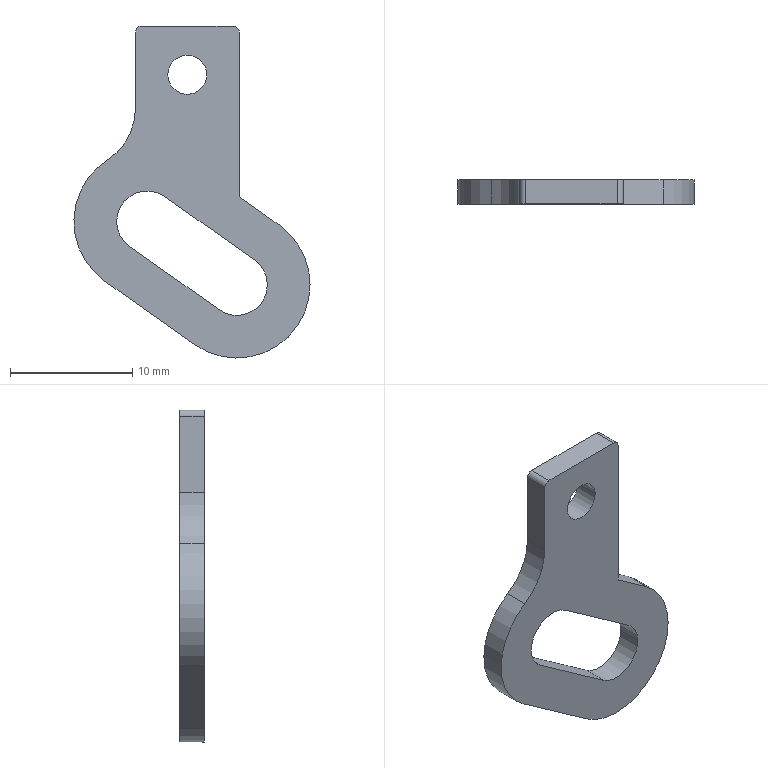Component | SolidWorks | CLS-MechanismOperatingAxisBracketAssembly.SLDPRT-1_CLS-MechanismPositioningSlide-1 | 1 solid | 20 faces | box 19.35 x 2 x 27.21 mm | volume 493 mm3 | cylinder 11 | plane 9 | commonest cylinder face diameters 5 x3 12 x3 3.2 x2 1 x2 10 x1
STEP:
#1=COLOUR_RGB('',0.7922,0.8196,0.9333);
#2=FILL_AREA_STYLE_COLOUR('',#1);
#3=FILL_AREA_STYLE('',(#2));
#4=SURFACE_STYLE_FILL_AREA(#3);
#5=SURFACE_SIDE_STYLE('',(#4));
#6=SURFACE_STYLE_USAGE(.BOTH.,#5);
#7=PRESENTATION_STYLE_ASSIGNMENT((#6));
#8=CARTESIAN_POINT('',(-2.391,-0.8783,-2.185));
#9=VERTEX_POINT('',#8);
#10=CARTESIAN_POINT('',(-2.265,-0.8783,-2.185));
#11=VERTEX_POINT('',#10);
#12=CARTESIAN_POINT('',(-2.328,-0.8783,-2.185));
#13=DIRECTION('',(0.,1.,-0.));
#14=DIRECTION('',(1.,0.,0.));
#15=AXIS2_PLACEMENT_3D('',#12,#13,#14);
#16=CIRCLE('',#15,0.06299);
#17=EDGE_CURVE('',#9,#11,#16,.T.);
#18=ORIENTED_EDGE('',*,*,#17,.F.);
#19=CARTESIAN_POINT('',(-2.391,-0.7995,-2.185));
#20=VERTEX_POINT('',#19);
#21=CARTESIAN_POINT('',(-2.391,-0.8783,-2.185));
#22=DIRECTION('',(0.,1.,-0.));
#23=VECTOR('',#22,39.37);
#24=LINE('',#21,#23);
#25=EDGE_CURVE('',#9,#20,#24,.T.);
#26=ORIENTED_EDGE('',*,*,#25,.T.);
#27=CARTESIAN_POINT('',(-2.265,-0.7995,-2.185));
#28=VERTEX_POINT('',#27);
#29=CARTESIAN_POINT('',(-2.328,-0.7995,-2.185));
#30=DIRECTION('',(0.,1.,-0.));
#31=DIRECTION('',(1.,0.,0.));
#32=AXIS2_PLACEMENT_3D('',#29,#30,#31);
#33=CIRCLE('',#32,0.06299);
#34=EDGE_CURVE('',#20,#28,#33,.T.);
#35=ORIENTED_EDGE('',*,*,#34,.T.);
#36=CARTESIAN_POINT('',(-2.265,-0.8783,-2.185));
#37=DIRECTION('',(0.,1.,-0.));
#38=VECTOR('',#37,39.37);
#39=LINE('',#36,#38);
#40=EDGE_CURVE('',#11,#28,#39,.T.);
#41=ORIENTED_EDGE('',*,*,#40,.F.);
#42=EDGE_LOOP('',(#18,#26,#35,#41));
#43=FACE_OUTER_BOUND('',#42,.T.);
#44=CARTESIAN_POINT('',(-2.328,-0.8783,-2.185));
#45=DIRECTION('',(0.,1.,-0.));
#46=DIRECTION('',(1.,0.,0.));
#47=AXIS2_PLACEMENT_3D('',#44,#45,#46);
#48=CYLINDRICAL_SURFACE('',#47,0.06299);
#49=ADVANCED_FACE('',(#43),#48,.F.);
#50=CARTESIAN_POINT('',(-2.07,-0.8783,-2.862));
#51=VERTEX_POINT('',#50);
#52=CARTESIAN_POINT('',(-2.225,-0.8783,-2.943));
#53=VERTEX_POINT('',#52);
#54=CARTESIAN_POINT('',(-2.168,-0.8783,-2.862));
#55=DIRECTION('',(0.,1.,-0.));
#56=DIRECTION('',(1.,0.,0.));
#57=AXIS2_PLACEMENT_3D('',#54,#55,#56);
#58=CIRCLE('',#57,0.09843);
#59=EDGE_CURVE('',#51,#53,#58,.T.);
#60=ORIENTED_EDGE('',*,*,#59,.F.);
#61=CARTESIAN_POINT('',(-2.07,-0.7995,-2.862));
#62=VERTEX_POINT('',#61);
#63=CARTESIAN_POINT('',(-2.07,-0.8783,-2.862));
#64=DIRECTION('',(0.,1.,-0.));
#65=VECTOR('',#64,39.37);
#66=LINE('',#63,#65);
#67=EDGE_CURVE('',#51,#62,#66,.T.);
#68=ORIENTED_EDGE('',*,*,#67,.T.);
#69=CARTESIAN_POINT('',(-2.225,-0.7995,-2.943));
#70=VERTEX_POINT('',#69);
#71=CARTESIAN_POINT('',(-2.168,-0.7995,-2.862));
#72=DIRECTION('',(0.,1.,-0.));
#73=DIRECTION('',(1.,0.,0.));
#74=AXIS2_PLACEMENT_3D('',#71,#72,#73);
#75=CIRCLE('',#74,0.09843);
#76=EDGE_CURVE('',#62,#70,#75,.T.);
#77=ORIENTED_EDGE('',*,*,#76,.T.);
#78=CARTESIAN_POINT('',(-2.225,-0.8783,-2.943));
#79=DIRECTION('',(0.,1.,-0.));
#80=VECTOR('',#79,39.37);
#81=LINE('',#78,#80);
#82=EDGE_CURVE('',#53,#70,#81,.T.);
#83=ORIENTED_EDGE('',*,*,#82,.F.);
#84=EDGE_LOOP('',(#60,#68,#77,#83));
#85=FACE_OUTER_BOUND('',#84,.T.);
#86=CARTESIAN_POINT('',(-2.168,-0.8783,-2.862));
#87=DIRECTION('',(0.,1.,-0.));
#88=DIRECTION('',(1.,0.,0.));
#89=AXIS2_PLACEMENT_3D('',#86,#87,#88);
#90=CYLINDRICAL_SURFACE('',#89,0.09843);
#91=ADVANCED_FACE('',(#85),#90,.F.);
#92=CARTESIAN_POINT('',(-2.032,-0.8783,-2.669));
#93=VERTEX_POINT('',#92);
#94=CARTESIAN_POINT('',(-1.932,-0.8783,-2.862));
#95=VERTEX_POINT('',#94);
#96=CARTESIAN_POINT('',(-2.168,-0.8783,-2.862));
#97=DIRECTION('',(0.,1.,-0.));
#98=DIRECTION('',(1.,0.,0.));
#99=AXIS2_PLACEMENT_3D('',#96,#97,#98);
#100=CIRCLE('',#99,0.2362);
#101=EDGE_CURVE('',#93,#95,#100,.T.);
#102=ORIENTED_EDGE('',*,*,#101,.T.);
#103=CARTESIAN_POINT('',(-1.932,-0.7995,-2.862));
#104=VERTEX_POINT('',#103);
#105=CARTESIAN_POINT('',(-1.932,-0.8783,-2.862));
#106=DIRECTION('',(0.,1.,-0.));
#107=VECTOR('',#106,39.37);
#108=LINE('',#105,#107);
#109=EDGE_CURVE('',#95,#104,#108,.T.);
#110=ORIENTED_EDGE('',*,*,#109,.T.);
#111=CARTESIAN_POINT('',(-2.032,-0.7995,-2.669));
#112=VERTEX_POINT('',#111);
#113=CARTESIAN_POINT('',(-2.168,-0.7995,-2.862));
#114=DIRECTION('',(0.,1.,-0.));
#115=DIRECTION('',(1.,0.,0.));
#116=AXIS2_PLACEMENT_3D('',#113,#114,#115);
#117=CIRCLE('',#116,0.2362);
#118=EDGE_CURVE('',#112,#104,#117,.T.);
#119=ORIENTED_EDGE('',*,*,#118,.F.);
#120=CARTESIAN_POINT('',(-2.032,-0.8783,-2.669));
#121=DIRECTION('',(0.,1.,-0.));
#122=VECTOR('',#121,39.37);
#123=LINE('',#120,#122);
#124=EDGE_CURVE('',#93,#112,#123,.T.);
#125=ORIENTED_EDGE('',*,*,#124,.F.);
#126=EDGE_LOOP('',(#102,#110,#119,#125));
#127=FACE_OUTER_BOUND('',#126,.T.);
#128=CARTESIAN_POINT('',(-2.168,-0.8783,-2.862));
#129=DIRECTION('',(0.,1.,-0.));
#130=DIRECTION('',(1.,0.,0.));
#131=AXIS2_PLACEMENT_3D('',#128,#129,#130);
#132=CYLINDRICAL_SURFACE('',#131,0.2362);
#133=ADVANCED_FACE('',(#127),#132,.T.);
#134=CARTESIAN_POINT('',(-2.495,-0.8783,-2.294));
#135=VERTEX_POINT('',#134);
#136=CARTESIAN_POINT('',(-2.495,-0.8783,-2.047));
#137=VERTEX_POINT('',#136);
#138=CARTESIAN_POINT('',(-2.495,-0.8783,-2.425));
#139=DIRECTION('',(0.,0.,1.));
#140=VECTOR('',#139,39.37);
#141=LINE('',#138,#140);
#142=EDGE_CURVE('',#135,#137,#141,.T.);
#143=ORIENTED_EDGE('',*,*,#142,.T.);
#144=CARTESIAN_POINT('',(-2.495,-0.7995,-2.047));
#145=VERTEX_POINT('',#144);
#146=CARTESIAN_POINT('',(-2.495,-0.8783,-2.047));
#147=DIRECTION('',(0.,1.,-0.));
#148=VECTOR('',#147,39.37);
#149=LINE('',#146,#148);
#150=EDGE_CURVE('',#137,#145,#149,.T.);
#151=ORIENTED_EDGE('',*,*,#150,.T.);
#152=CARTESIAN_POINT('',(-2.495,-0.7995,-2.294));
#153=VERTEX_POINT('',#152);
#154=CARTESIAN_POINT('',(-2.495,-0.7995,-2.425));
#155=DIRECTION('',(0.,0.,1.));
#156=VECTOR('',#155,39.37);
#157=LINE('',#154,#156);
#158=EDGE_CURVE('',#153,#145,#157,.T.);
#159=ORIENTED_EDGE('',*,*,#158,.F.);
#160=CARTESIAN_POINT('',(-2.495,-0.8783,-2.294));
#161=DIRECTION('',(-0.,-1.,0.));
#162=VECTOR('',#161,39.37);
#163=LINE('',#160,#162);
#164=EDGE_CURVE('',#153,#135,#163,.T.);
#165=ORIENTED_EDGE('',*,*,#164,.T.);
#166=EDGE_LOOP('',(#143,#151,#159,#165));
#167=FACE_OUTER_BOUND('',#166,.T.);
#168=CARTESIAN_POINT('',(-2.495,-0.8783,-2.425));
#169=DIRECTION('',(-1.,0.,0.));
#170=DIRECTION('',(0.,1.,-0.));
#171=AXIS2_PLACEMENT_3D('',#168,#169,#170);
#172=PLANE('',#171);
#173=ADVANCED_FACE('',(#167),#172,.T.);
#174=CARTESIAN_POINT('',(-2.594,-0.8783,-2.851));
#175=VERTEX_POINT('',#174);
#176=CARTESIAN_POINT('',(-2.585,-0.8783,-2.459));
#177=VERTEX_POINT('',#176);
#178=CARTESIAN_POINT('',(-2.458,-0.8783,-2.658));
#179=DIRECTION('',(0.,1.,-0.));
#180=DIRECTION('',(1.,0.,0.));
#181=AXIS2_PLACEMENT_3D('',#178,#179,#180);
#182=CIRCLE('',#181,0.2362);
#183=EDGE_CURVE('',#175,#177,#182,.T.);
#184=ORIENTED_EDGE('',*,*,#183,.T.);
#185=CARTESIAN_POINT('',(-2.585,-0.7995,-2.459));
#186=VERTEX_POINT('',#185);
#187=CARTESIAN_POINT('',(-2.585,-0.8783,-2.459));
#188=DIRECTION('',(0.,1.,-0.));
#189=VECTOR('',#188,39.37);
#190=LINE('',#187,#189);
#191=EDGE_CURVE('',#177,#186,#190,.T.);
#192=ORIENTED_EDGE('',*,*,#191,.T.);
#193=CARTESIAN_POINT('',(-2.594,-0.7995,-2.851));
#194=VERTEX_POINT('',#193);
#195=CARTESIAN_POINT('',(-2.458,-0.7995,-2.658));
#196=DIRECTION('',(0.,1.,-0.));
#197=DIRECTION('',(1.,0.,0.));
#198=AXIS2_PLACEMENT_3D('',#195,#196,#197);
#199=CIRCLE('',#198,0.2362);
#200=EDGE_CURVE('',#194,#186,#199,.T.);
#201=ORIENTED_EDGE('',*,*,#200,.F.);
#202=CARTESIAN_POINT('',(-2.594,-0.8783,-2.851));
#203=DIRECTION('',(0.,1.,-0.));
#204=VECTOR('',#203,39.37);
#205=LINE('',#202,#204);
#206=EDGE_CURVE('',#175,#194,#205,.T.);
#207=ORIENTED_EDGE('',*,*,#206,.F.);
#208=EDGE_LOOP('',(#184,#192,#201,#207));
#209=FACE_OUTER_BOUND('',#208,.T.);
#210=CARTESIAN_POINT('',(-2.458,-0.8783,-2.658));
#211=DIRECTION('',(0.,1.,-0.));
#212=DIRECTION('',(1.,0.,0.));
#213=AXIS2_PLACEMENT_3D('',#210,#211,#212);
#214=CYLINDRICAL_SURFACE('',#213,0.2362);
#215=ADVANCED_FACE('',(#209),#214,.T.);
#216=CARTESIAN_POINT('',(-2.304,-0.7995,-3.055));
#217=VERTEX_POINT('',#216);
#218=CARTESIAN_POINT('',(-2.594,-0.7995,-2.851));
#219=DIRECTION('',(-0.817,0.,0.5767));
#220=VECTOR('',#219,39.37);
#221=LINE('',#218,#220);
#222=EDGE_CURVE('',#217,#194,#221,.T.);
#223=ORIENTED_EDGE('',*,*,#222,.F.);
#224=CARTESIAN_POINT('',(-2.304,-0.8783,-3.055));
#225=VERTEX_POINT('',#224);
#226=CARTESIAN_POINT('',(-2.304,-0.8783,-3.055));
#227=DIRECTION('',(0.,1.,-0.));
#228=VECTOR('',#227,39.37);
#229=LINE('',#226,#228);
#230=EDGE_CURVE('',#225,#217,#229,.T.);
#231=ORIENTED_EDGE('',*,*,#230,.F.);
#232=CARTESIAN_POINT('',(-2.594,-0.8783,-2.851));
#233=DIRECTION('',(-0.817,0.,0.5767));
#234=VECTOR('',#233,39.37);
#235=LINE('',#232,#234);
#236=EDGE_CURVE('',#225,#175,#235,.T.);
#237=ORIENTED_EDGE('',*,*,#236,.T.);
#238=ORIENTED_EDGE('',*,*,#206,.T.);
#239=EDGE_LOOP('',(#223,#231,#237,#238));
#240=FACE_OUTER_BOUND('',#239,.T.);
#241=CARTESIAN_POINT('',(-2.594,-0.8783,-2.851));
#242=DIRECTION('',(-0.5767,-0.,-0.817));
#243=DIRECTION('',(-0.817,0.,0.5767));
#244=AXIS2_PLACEMENT_3D('',#241,#242,#243);
#245=PLANE('',#244);
#246=ADVANCED_FACE('',(#240),#245,.T.);
#247=ORIENTED_EDGE('',*,*,#109,.F.);
#248=CARTESIAN_POINT('',(-2.168,-0.8783,-2.862));
#249=DIRECTION('',(0.,1.,-0.));
#250=DIRECTION('',(1.,0.,0.));
#251=AXIS2_PLACEMENT_3D('',#248,#249,#250);
#252=CIRCLE('',#251,0.2362);
#253=EDGE_CURVE('',#95,#225,#252,.T.);
#254=ORIENTED_EDGE('',*,*,#253,.T.);
#255=ORIENTED_EDGE('',*,*,#230,.T.);
#256=CARTESIAN_POINT('',(-2.168,-0.7995,-2.862));
#257=DIRECTION('',(0.,1.,-0.));
#258=DIRECTION('',(1.,0.,0.));
#259=AXIS2_PLACEMENT_3D('',#256,#257,#258);
#260=CIRCLE('',#259,0.2362);
#261=EDGE_CURVE('',#104,#217,#260,.T.);
#262=ORIENTED_EDGE('',*,*,#261,.F.);
#263=EDGE_LOOP('',(#247,#254,#255,#262));
#264=FACE_OUTER_BOUND('',#263,.T.);
#265=CARTESIAN_POINT('',(-2.168,-0.8783,-2.862));
#266=DIRECTION('',(0.,1.,-0.));
#267=DIRECTION('',(1.,0.,0.));
#268=AXIS2_PLACEMENT_3D('',#265,#266,#267);
#269=CYLINDRICAL_SURFACE('',#268,0.2362);
#270=ADVANCED_FACE('',(#264),#269,.T.);
#271=CARTESIAN_POINT('',(-2.161,-0.7995,-2.578));
#272=VERTEX_POINT('',#271);
#273=CARTESIAN_POINT('',(-2.161,-0.7995,-2.578));
#274=DIRECTION('',(0.817,-0.,-0.5767));
#275=VECTOR('',#274,39.37);
#276=LINE('',#273,#275);
#277=EDGE_CURVE('',#272,#112,#276,.T.);
#278=ORIENTED_EDGE('',*,*,#277,.F.);
#279=CARTESIAN_POINT('',(-2.161,-0.8783,-2.578));
#280=VERTEX_POINT('',#279);
#281=CARTESIAN_POINT('',(-2.161,-0.8783,-2.578));
#282=DIRECTION('',(0.,1.,-0.));
#283=VECTOR('',#282,39.37);
#284=LINE('',#281,#283);
#285=EDGE_CURVE('',#280,#272,#284,.T.);
#286=ORIENTED_EDGE('',*,*,#285,.F.);
#287=CARTESIAN_POINT('',(-2.161,-0.8783,-2.578));
#288=DIRECTION('',(0.817,-0.,-0.5767));
#289=VECTOR('',#288,39.37);
#290=LINE('',#287,#289);
#291=EDGE_CURVE('',#280,#93,#290,.T.);
#292=ORIENTED_EDGE('',*,*,#291,.T.);
#293=ORIENTED_EDGE('',*,*,#124,.T.);
#294=EDGE_LOOP('',(#278,#286,#292,#293));
#295=FACE_OUTER_BOUND('',#294,.T.);
#296=CARTESIAN_POINT('',(-2.161,-0.8783,-2.578));
#297=DIRECTION('',(0.5767,0.,0.817));
#298=DIRECTION('',(0.817,-0.,-0.5767));
#299=AXIS2_PLACEMENT_3D('',#296,#297,#298);
#300=PLANE('',#299);
#301=ADVANCED_FACE('',(#295),#300,.T.);
#302=CARTESIAN_POINT('',(-2.161,-0.7995,-2.047));
#303=VERTEX_POINT('',#302);
#304=CARTESIAN_POINT('',(-2.161,-0.7995,-2.027));
#305=DIRECTION('',(-0.,-0.,-1.));
#306=VECTOR('',#305,39.37);
#307=LINE('',#304,#306);
#308=EDGE_CURVE('',#303,#272,#307,.T.);
#309=ORIENTED_EDGE('',*,*,#308,.F.);
#310=CARTESIAN_POINT('',(-2.161,-0.8783,-2.047));
#311=VERTEX_POINT('',#310);
#312=CARTESIAN_POINT('',(-2.161,-0.8783,-2.047));
#313=DIRECTION('',(-0.,-1.,0.));
#314=VECTOR('',#313,39.37);
#315=LINE('',#312,#314);
#316=EDGE_CURVE('',#303,#311,#315,.T.);
#317=ORIENTED_EDGE('',*,*,#316,.T.);
#318=CARTESIAN_POINT('',(-2.161,-0.8783,-2.027));
#319=DIRECTION('',(-0.,-0.,-1.));
#320=VECTOR('',#319,39.37);
#321=LINE('',#318,#320);
#322=EDGE_CURVE('',#311,#280,#321,.T.);
#323=ORIENTED_EDGE('',*,*,#322,.T.);
#324=ORIENTED_EDGE('',*,*,#285,.T.);
#325=EDGE_LOOP('',(#309,#317,#323,#324));
#326=FACE_OUTER_BOUND('',#325,.T.);
#327=CARTESIAN_POINT('',(-2.161,-0.8783,-2.027));
#328=DIRECTION('',(1.,-0.,-0.));
#329=DIRECTION('',(-0.,-1.,0.));
#330=AXIS2_PLACEMENT_3D('',#327,#328,#329);
#331=PLANE('',#330);
#332=ADVANCED_FACE('',(#326),#331,.T.);
#333=CARTESIAN_POINT('',(-2.475,-0.7995,-2.027));
#334=VERTEX_POINT('',#333);
#335=CARTESIAN_POINT('',(-2.18,-0.7995,-2.027));
#336=VERTEX_POINT('',#335);
#337=CARTESIAN_POINT('',(-2.495,-0.7995,-2.027));
#338=DIRECTION('',(1.,-0.,-0.));
#339=VECTOR('',#338,39.37);
#340=LINE('',#337,#339);
#341=EDGE_CURVE('',#334,#336,#340,.T.);
#342=ORIENTED_EDGE('',*,*,#341,.F.);
#343=CARTESIAN_POINT('',(-2.475,-0.8783,-2.027));
#344=VERTEX_POINT('',#343);
#345=CARTESIAN_POINT('',(-2.475,-0.8783,-2.027));
#346=DIRECTION('',(-0.,-1.,0.));
#347=VECTOR('',#346,39.37);
#348=LINE('',#345,#347);
#349=EDGE_CURVE('',#334,#344,#348,.T.);
#350=ORIENTED_EDGE('',*,*,#349,.T.);
#351=CARTESIAN_POINT('',(-2.18,-0.8783,-2.027));
#352=VERTEX_POINT('',#351);
#353=CARTESIAN_POINT('',(-2.495,-0.8783,-2.027));
#354=DIRECTION('',(1.,-0.,-0.));
#355=VECTOR('',#354,39.37);
#356=LINE('',#353,#355);
#357=EDGE_CURVE('',#344,#352,#356,.T.);
#358=ORIENTED_EDGE('',*,*,#357,.T.);
#359=CARTESIAN_POINT('',(-2.18,-0.8783,-2.027));
#360=DIRECTION('',(0.,1.,-0.));
#361=VECTOR('',#360,39.37);
#362=LINE('',#359,#361);
#363=EDGE_CURVE('',#352,#336,#362,.T.);
#364=ORIENTED_EDGE('',*,*,#363,.T.);
#365=EDGE_LOOP('',(#342,#350,#358,#364));
#366=FACE_OUTER_BOUND('',#365,.T.);
#367=CARTESIAN_POINT('',(-2.495,-0.8783,-2.027));
#368=DIRECTION('',(0.,0.,1.));
#369=DIRECTION('',(-0.,-1.,0.));
#370=AXIS2_PLACEMENT_3D('',#367,#368,#369);
#371=PLANE('',#370);
#372=ADVANCED_FACE('',(#366),#371,.T.);
#373=CARTESIAN_POINT('',(-2.328,-0.8783,-2.185));
#374=DIRECTION('',(0.,1.,-0.));
#375=DIRECTION('',(1.,0.,0.));
#376=AXIS2_PLACEMENT_3D('',#373,#374,#375);
#377=CIRCLE('',#376,0.06299);
#378=EDGE_CURVE('',#11,#9,#377,.T.);
#379=ORIENTED_EDGE('',*,*,#378,.T.);
#380=ORIENTED_EDGE('',*,*,#17,.T.);
#381=EDGE_LOOP('',(#379,#380));
#382=FACE_BOUND('',#381,.T.);
#383=CARTESIAN_POINT('',(-2.514,-0.8783,-2.738));
#384=VERTEX_POINT('',#383);
#385=CARTESIAN_POINT('',(-2.401,-0.8783,-2.577));
#386=VERTEX_POINT('',#385);
#387=CARTESIAN_POINT('',(-2.458,-0.8783,-2.658));
#388=DIRECTION('',(0.,1.,-0.));
#389=DIRECTION('',(1.,0.,0.));
#390=AXIS2_PLACEMENT_3D('',#387,#388,#389);
#391=CIRCLE('',#390,0.09843);
#392=EDGE_CURVE('',#384,#386,#391,.T.);
#393=ORIENTED_EDGE('',*,*,#392,.T.);
#394=CARTESIAN_POINT('',(-2.111,-0.8783,-2.782));
#395=VERTEX_POINT('',#394);
#396=CARTESIAN_POINT('',(-2.111,-0.8783,-2.782));
#397=DIRECTION('',(0.817,-0.,-0.5767));
#398=VECTOR('',#397,39.37);
#399=LINE('',#396,#398);
#400=EDGE_CURVE('',#386,#395,#399,.T.);
#401=ORIENTED_EDGE('',*,*,#400,.T.);
#402=CARTESIAN_POINT('',(-2.168,-0.8783,-2.862));
#403=DIRECTION('',(0.,1.,-0.));
#404=DIRECTION('',(1.,0.,0.));
#405=AXIS2_PLACEMENT_3D('',#402,#403,#404);
#406=CIRCLE('',#405,0.09843);
#407=EDGE_CURVE('',#395,#51,#406,.T.);
#408=ORIENTED_EDGE('',*,*,#407,.T.);
#409=ORIENTED_EDGE('',*,*,#59,.T.);
#410=CARTESIAN_POINT('',(-2.225,-0.8783,-2.943));
#411=DIRECTION('',(-0.817,0.,0.5767));
#412=VECTOR('',#411,39.37);
#413=LINE('',#410,#412);
#414=EDGE_CURVE('',#53,#384,#413,.T.);
#415=ORIENTED_EDGE('',*,*,#414,.T.);
#416=EDGE_LOOP('',(#393,#401,#408,#409,#415));
#417=FACE_BOUND('',#416,.T.);
#418=ORIENTED_EDGE('',*,*,#357,.F.);
#419=CARTESIAN_POINT('',(-2.475,-0.8783,-2.047));
#420=DIRECTION('',(-0.,-1.,0.));
#421=DIRECTION('',(1.,0.,0.));
#422=AXIS2_PLACEMENT_3D('',#419,#420,#421);
#423=CIRCLE('',#422,0.01969);
#424=EDGE_CURVE('',#344,#137,#423,.T.);
#425=ORIENTED_EDGE('',*,*,#424,.T.);
#426=ORIENTED_EDGE('',*,*,#142,.F.);
#427=CARTESIAN_POINT('',(-2.692,-0.8783,-2.294));
#428=DIRECTION('',(0.,1.,-0.));
#429=DIRECTION('',(1.,0.,0.));
#430=AXIS2_PLACEMENT_3D('',#427,#428,#429);
#431=CIRCLE('',#430,0.1969);
#432=EDGE_CURVE('',#135,#177,#431,.T.);
#433=ORIENTED_EDGE('',*,*,#432,.T.);
#434=ORIENTED_EDGE('',*,*,#183,.F.);
#435=ORIENTED_EDGE('',*,*,#236,.F.);
#436=ORIENTED_EDGE('',*,*,#253,.F.);
#437=ORIENTED_EDGE('',*,*,#101,.F.);
#438=ORIENTED_EDGE('',*,*,#291,.F.);
#439=ORIENTED_EDGE('',*,*,#322,.F.);
#440=CARTESIAN_POINT('',(-2.18,-0.8783,-2.047));
#441=DIRECTION('',(-0.,-1.,0.));
#442=DIRECTION('',(1.,0.,0.));
#443=AXIS2_PLACEMENT_3D('',#440,#441,#442);
#444=CIRCLE('',#443,0.01969);
#445=EDGE_CURVE('',#311,#352,#444,.T.);
#446=ORIENTED_EDGE('',*,*,#445,.T.);
#447=EDGE_LOOP('',(#418,#425,#426,#433,#434,#435,#436,#437,#438,#439,#446));
#448=FACE_OUTER_BOUND('',#447,.T.);
#449=CARTESIAN_POINT('',(-2.168,-0.8783,-2.862));
#450=DIRECTION('',(0.,1.,-0.));
#451=DIRECTION('',(1.,-0.,-0.));
#452=AXIS2_PLACEMENT_3D('',#449,#450,#451);
#453=PLANE('',#452);
#454=ADVANCED_FACE('',(#382,#417,#448),#453,.F.);
#455=CARTESIAN_POINT('',(-2.328,-0.7995,-2.185));
#456=DIRECTION('',(0.,1.,-0.));
#457=DIRECTION('',(1.,0.,0.));
#458=AXIS2_PLACEMENT_3D('',#455,#456,#457);
#459=CIRCLE('',#458,0.06299);
#460=EDGE_CURVE('',#28,#20,#459,.T.);
#461=ORIENTED_EDGE('',*,*,#460,.F.);
#462=ORIENTED_EDGE('',*,*,#34,.F.);
#463=EDGE_LOOP('',(#461,#462));
#464=FACE_BOUND('',#463,.T.);
#465=CARTESIAN_POINT('',(-2.401,-0.7995,-2.577));
#466=VERTEX_POINT('',#465);
#467=CARTESIAN_POINT('',(-2.111,-0.7995,-2.782));
#468=VERTEX_POINT('',#467);
#469=CARTESIAN_POINT('',(-2.111,-0.7995,-2.782));
#470=DIRECTION('',(0.817,-0.,-0.5767));
#471=VECTOR('',#470,39.37);
#472=LINE('',#469,#471);
#473=EDGE_CURVE('',#466,#468,#472,.T.);
#474=ORIENTED_EDGE('',*,*,#473,.F.);
#475=CARTESIAN_POINT('',(-2.514,-0.7995,-2.738));
#476=VERTEX_POINT('',#475);
#477=CARTESIAN_POINT('',(-2.458,-0.7995,-2.658));
#478=DIRECTION('',(0.,1.,-0.));
#479=DIRECTION('',(1.,0.,0.));
#480=AXIS2_PLACEMENT_3D('',#477,#478,#479);
#481=CIRCLE('',#480,0.09843);
#482=EDGE_CURVE('',#476,#466,#481,.T.);
#483=ORIENTED_EDGE('',*,*,#482,.F.);
#484=CARTESIAN_POINT('',(-2.225,-0.7995,-2.943));
#485=DIRECTION('',(-0.817,0.,0.5767));
#486=VECTOR('',#485,39.37);
#487=LINE('',#484,#486);
#488=EDGE_CURVE('',#70,#476,#487,.T.);
#489=ORIENTED_EDGE('',*,*,#488,.F.);
#490=ORIENTED_EDGE('',*,*,#76,.F.);
#491=CARTESIAN_POINT('',(-2.168,-0.7995,-2.862));
#492=DIRECTION('',(0.,1.,-0.));
#493=DIRECTION('',(1.,0.,0.));
#494=AXIS2_PLACEMENT_3D('',#491,#492,#493);
#495=CIRCLE('',#494,0.09843);
#496=EDGE_CURVE('',#468,#62,#495,.T.);
#497=ORIENTED_EDGE('',*,*,#496,.F.);
#498=EDGE_LOOP('',(#474,#483,#489,#490,#497));
#499=FACE_BOUND('',#498,.T.);
#500=ORIENTED_EDGE('',*,*,#158,.T.);
#501=CARTESIAN_POINT('',(-2.475,-0.7995,-2.047));
#502=DIRECTION('',(0.,1.,-0.));
#503=DIRECTION('',(1.,0.,0.));
#504=AXIS2_PLACEMENT_3D('',#501,#502,#503);
#505=CIRCLE('',#504,0.01969);
#506=EDGE_CURVE('',#145,#334,#505,.T.);
#507=ORIENTED_EDGE('',*,*,#506,.T.);
#508=ORIENTED_EDGE('',*,*,#341,.T.);
#509=CARTESIAN_POINT('',(-2.18,-0.7995,-2.047));
#510=DIRECTION('',(0.,1.,-0.));
#511=DIRECTION('',(1.,0.,0.));
#512=AXIS2_PLACEMENT_3D('',#509,#510,#511);
#513=CIRCLE('',#512,0.01969);
#514=EDGE_CURVE('',#336,#303,#513,.T.);
#515=ORIENTED_EDGE('',*,*,#514,.T.);
#516=ORIENTED_EDGE('',*,*,#308,.T.);
#517=ORIENTED_EDGE('',*,*,#277,.T.);
#518=ORIENTED_EDGE('',*,*,#118,.T.);
#519=ORIENTED_EDGE('',*,*,#261,.T.);
#520=ORIENTED_EDGE('',*,*,#222,.T.);
#521=ORIENTED_EDGE('',*,*,#200,.T.);
#522=CARTESIAN_POINT('',(-2.692,-0.7995,-2.294));
#523=DIRECTION('',(-0.,-1.,0.));
#524=DIRECTION('',(1.,0.,0.));
#525=AXIS2_PLACEMENT_3D('',#522,#523,#524);
#526=CIRCLE('',#525,0.1969);
#527=EDGE_CURVE('',#186,#153,#526,.T.);
#528=ORIENTED_EDGE('',*,*,#527,.T.);
#529=EDGE_LOOP('',(#500,#507,#508,#515,#516,#517,#518,#519,#520,#521,#528));
#530=FACE_OUTER_BOUND('',#529,.T.);
#531=CARTESIAN_POINT('',(-2.168,-0.7995,-2.862));
#532=DIRECTION('',(0.,1.,-0.));
#533=DIRECTION('',(1.,-0.,-0.));
#534=AXIS2_PLACEMENT_3D('',#531,#532,#533);
#535=PLANE('',#534);
#536=ADVANCED_FACE('',(#464,#499,#530),#535,.T.);
#537=ORIENTED_EDGE('',*,*,#473,.T.);
#538=CARTESIAN_POINT('',(-2.111,-0.8783,-2.782));
#539=DIRECTION('',(0.,1.,-0.));
#540=VECTOR('',#539,39.37);
#541=LINE('',#538,#540);
#542=EDGE_CURVE('',#395,#468,#541,.T.);
#543=ORIENTED_EDGE('',*,*,#542,.F.);
#544=ORIENTED_EDGE('',*,*,#400,.F.);
#545=CARTESIAN_POINT('',(-2.401,-0.8783,-2.577));
#546=DIRECTION('',(0.,1.,-0.));
#547=VECTOR('',#546,39.37);
#548=LINE('',#545,#547);
#549=EDGE_CURVE('',#386,#466,#548,.T.);
#550=ORIENTED_EDGE('',*,*,#549,.T.);
#551=EDGE_LOOP('',(#537,#543,#544,#550));
#552=FACE_OUTER_BOUND('',#551,.T.);
#553=CARTESIAN_POINT('',(-2.111,-0.8783,-2.782));
#554=DIRECTION('',(0.5767,0.,0.817));
#555=DIRECTION('',(0.817,-0.,-0.5767));
#556=AXIS2_PLACEMENT_3D('',#553,#554,#555);
#557=PLANE('',#556);
#558=ADVANCED_FACE('',(#552),#557,.F.);
#559=ORIENTED_EDGE('',*,*,#482,.T.);
#560=ORIENTED_EDGE('',*,*,#549,.F.);
#561=ORIENTED_EDGE('',*,*,#392,.F.);
#562=CARTESIAN_POINT('',(-2.514,-0.8783,-2.738));
#563=DIRECTION('',(0.,1.,-0.));
#564=VECTOR('',#563,39.37);
#565=LINE('',#562,#564);
#566=EDGE_CURVE('',#384,#476,#565,.T.);
#567=ORIENTED_EDGE('',*,*,#566,.T.);
#568=EDGE_LOOP('',(#559,#560,#561,#567));
#569=FACE_OUTER_BOUND('',#568,.T.);
#570=CARTESIAN_POINT('',(-2.458,-0.8783,-2.658));
#571=DIRECTION('',(0.,1.,-0.));
#572=DIRECTION('',(1.,0.,0.));
#573=AXIS2_PLACEMENT_3D('',#570,#571,#572);
#574=CYLINDRICAL_SURFACE('',#573,0.09843);
#575=ADVANCED_FACE('',(#569),#574,.F.);
#576=ORIENTED_EDGE('',*,*,#488,.T.);
#577=ORIENTED_EDGE('',*,*,#566,.F.);
#578=ORIENTED_EDGE('',*,*,#414,.F.);
#579=ORIENTED_EDGE('',*,*,#82,.T.);
#580=EDGE_LOOP('',(#576,#577,#578,#579));
#581=FACE_OUTER_BOUND('',#580,.T.);
#582=CARTESIAN_POINT('',(-2.225,-0.8783,-2.943));
#583=DIRECTION('',(-0.5767,-0.,-0.817));
#584=DIRECTION('',(-0.817,0.,0.5767));
#585=AXIS2_PLACEMENT_3D('',#582,#583,#584);
#586=PLANE('',#585);
#587=ADVANCED_FACE('',(#581),#586,.F.);
#588=ORIENTED_EDGE('',*,*,#67,.F.);
#589=ORIENTED_EDGE('',*,*,#407,.F.);
#590=ORIENTED_EDGE('',*,*,#542,.T.);
#591=ORIENTED_EDGE('',*,*,#496,.T.);
#592=EDGE_LOOP('',(#588,#589,#590,#591));
#593=FACE_OUTER_BOUND('',#592,.T.);
#594=CARTESIAN_POINT('',(-2.168,-0.8783,-2.862));
#595=DIRECTION('',(0.,1.,-0.));
#596=DIRECTION('',(1.,0.,0.));
#597=AXIS2_PLACEMENT_3D('',#594,#595,#596);
#598=CYLINDRICAL_SURFACE('',#597,0.09843);
#599=ADVANCED_FACE('',(#593),#598,.F.);
#600=ORIENTED_EDGE('',*,*,#432,.F.);
#601=ORIENTED_EDGE('',*,*,#164,.F.);
#602=ORIENTED_EDGE('',*,*,#527,.F.);
#603=ORIENTED_EDGE('',*,*,#191,.F.);
#604=EDGE_LOOP('',(#600,#601,#602,#603));
#605=FACE_OUTER_BOUND('',#604,.T.);
#606=CARTESIAN_POINT('',(-2.692,-0.8783,-2.294));
#607=DIRECTION('',(0.,1.,-0.));
#608=DIRECTION('',(1.,0.,0.));
#609=AXIS2_PLACEMENT_3D('',#606,#607,#608);
#610=CYLINDRICAL_SURFACE('',#609,0.1969);
#611=ADVANCED_FACE('',(#605),#610,.F.);
#612=ORIENTED_EDGE('',*,*,#25,.F.);
#613=ORIENTED_EDGE('',*,*,#378,.F.);
#614=ORIENTED_EDGE('',*,*,#40,.T.);
#615=ORIENTED_EDGE('',*,*,#460,.T.);
#616=EDGE_LOOP('',(#612,#613,#614,#615));
#617=FACE_OUTER_BOUND('',#616,.T.);
#618=CARTESIAN_POINT('',(-2.328,-0.8783,-2.185));
#619=DIRECTION('',(0.,1.,-0.));
#620=DIRECTION('',(1.,0.,0.));
#621=AXIS2_PLACEMENT_3D('',#618,#619,#620);
#622=CYLINDRICAL_SURFACE('',#621,0.06299);
#623=ADVANCED_FACE('',(#617),#622,.F.);
#624=ORIENTED_EDGE('',*,*,#424,.F.);
#625=ORIENTED_EDGE('',*,*,#349,.F.);
#626=ORIENTED_EDGE('',*,*,#506,.F.);
#627=ORIENTED_EDGE('',*,*,#150,.F.);
#628=EDGE_LOOP('',(#624,#625,#626,#627));
#629=FACE_OUTER_BOUND('',#628,.T.);
#630=CARTESIAN_POINT('',(-2.475,-0.8783,-2.047));
#631=DIRECTION('',(0.,1.,-0.));
#632=DIRECTION('',(1.,0.,0.));
#633=AXIS2_PLACEMENT_3D('',#630,#631,#632);
#634=CYLINDRICAL_SURFACE('',#633,0.01969);
#635=ADVANCED_FACE('',(#629),#634,.T.);
#636=ORIENTED_EDGE('',*,*,#445,.F.);
#637=ORIENTED_EDGE('',*,*,#316,.F.);
#638=ORIENTED_EDGE('',*,*,#514,.F.);
#639=ORIENTED_EDGE('',*,*,#363,.F.);
#640=EDGE_LOOP('',(#636,#637,#638,#639));
#641=FACE_OUTER_BOUND('',#640,.T.);
#642=CARTESIAN_POINT('',(-2.18,-0.8783,-2.047));
#643=DIRECTION('',(0.,1.,-0.));
#644=DIRECTION('',(1.,0.,0.));
#645=AXIS2_PLACEMENT_3D('',#642,#643,#644);
#646=CYLINDRICAL_SURFACE('',#645,0.01969);
#647=ADVANCED_FACE('',(#641),#646,.T.);
#648=CLOSED_SHELL('',(#49,#91,#133,#173,#215,#246,#270,#301,#332,#372,#454,#536,#558,#575,#587,#599,#611,#623,#635,#647));
#649=MANIFOLD_SOLID_BREP('',#648);
#650=STYLED_ITEM('',(#7),#649);
#651=(LENGTH_UNIT()NAMED_UNIT(*)SI_UNIT($,.METRE.));
#652=LENGTH_MEASURE_WITH_UNIT(LENGTH_MEASURE(0.0254),#651);
#653=DIMENSIONAL_EXPONENTS(1.,0.,0.,0.,0.,0.,0.);
#654=(CONVERSION_BASED_UNIT('',#652)LENGTH_UNIT()NAMED_UNIT(#653));
#655=UNCERTAINTY_MEASURE_WITH_UNIT(LENGTH_MEASURE(0.00001),#654,'','');
#656=(NAMED_UNIT(*)PLANE_ANGLE_UNIT()SI_UNIT($,.RADIAN.));
#657=(NAMED_UNIT(*)SI_UNIT($,.STERADIAN.)SOLID_ANGLE_UNIT());
#658=(GEOMETRIC_REPRESENTATION_CONTEXT(3)GLOBAL_UNCERTAINTY_ASSIGNED_CONTEXT((#655))GLOBAL_UNIT_ASSIGNED_CONTEXT((#654,#656,#657))REPRESENTATION_CONTEXT('',''));
#659=MECHANICAL_DESIGN_GEOMETRIC_PRESENTATION_REPRESENTATION('',(#650),#658);
#660=CARTESIAN_POINT('',(0.,0.,0.));
#661=DIRECTION('',(0.,0.,1.));
#662=DIRECTION('',(1.,0.,0.));
#663=AXIS2_PLACEMENT_3D('',#660,#661,#662);
#664=(LENGTH_UNIT()NAMED_UNIT(*)SI_UNIT($,.METRE.));
#665=LENGTH_MEASURE_WITH_UNIT(LENGTH_MEASURE(0.0254),#664);
#666=DIMENSIONAL_EXPONENTS(1.,0.,0.,0.,0.,0.,0.);
#667=(CONVERSION_BASED_UNIT('',#665)LENGTH_UNIT()NAMED_UNIT(#666));
#668=UNCERTAINTY_MEASURE_WITH_UNIT(LENGTH_MEASURE(0.00001),#667,'','');
#669=(NAMED_UNIT(*)PLANE_ANGLE_UNIT()SI_UNIT($,.RADIAN.));
#670=(NAMED_UNIT(*)SI_UNIT($,.STERADIAN.)SOLID_ANGLE_UNIT());
#671=(GEOMETRIC_REPRESENTATION_CONTEXT(3)GLOBAL_UNCERTAINTY_ASSIGNED_CONTEXT((#668))GLOBAL_UNIT_ASSIGNED_CONTEXT((#667,#669,#670))REPRESENTATION_CONTEXT('',''));
#672=ADVANCED_BREP_SHAPE_REPRESENTATION('',(#649,#663),#671);
#673=PRESENTATION_LAYER_ASSIGNMENT('','',(#650));